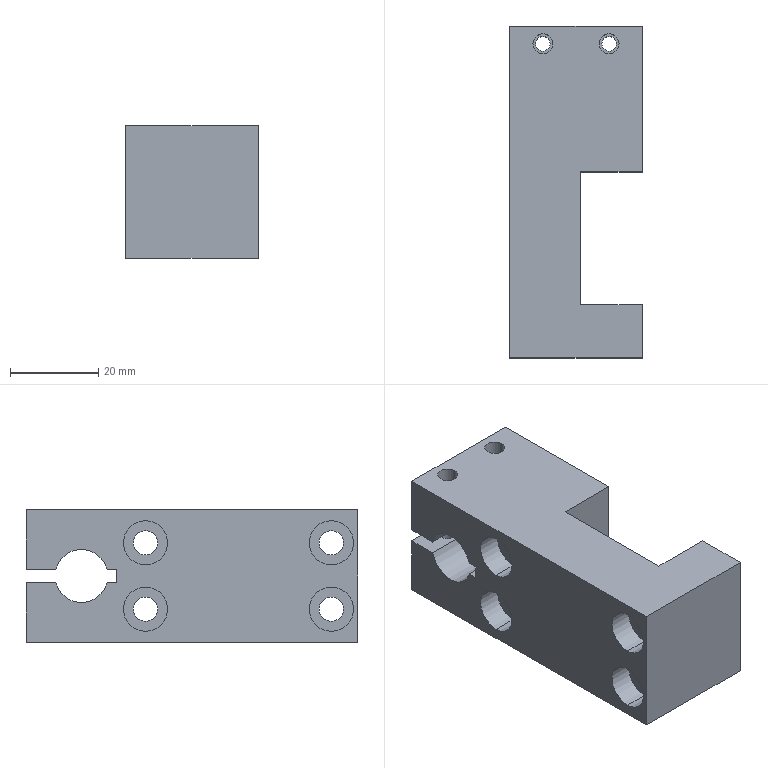Component | SolidWorks | XM-WST05-2005-1 | 1 solid | 46 faces | box 30 x 75 x 30 mm | volume 46036 mm3 | cylinder 26 | plane 20 | commonest cylinder face diameters 10 x8 5.5 x8 3.3 x4 4.5 x4 12 x2
build123d program:
from build123d import *

# Parameters (mm, degrees)
SKETCH1_W                                       = 30
SKETCH1_H                                       = 75
BOSS_EXTRUDE1_DEPTH                             = 15
SKETCH2_R                                       = 6
CUT_EXTRUDE1_DEPTH                              = 71.931
SKETCH4_W                                       = 3
SKETCH4_H                                       = 41
CUT_EXTRUDE3_DEPTH                              = 71.931
SKETCH11_W                                      = 30
SKETCH11_H                                      = 30
CUT_EXTRUDE6_DEPTH                              = 14
M5_HEX_SOCKET_HEAD_CAP_SCREW_CBORE2_D           = 5.5
M5_HEX_SOCKET_HEAD_CAP_SCREW_CBORE2_CBORE_D     = 10
M5_HEX_SOCKET_HEAD_CAP_SCREW_CBORE2_CBORE_DEPTH = 5.4
SKETCH17_R                                      = 2.25
CUT_EXTRUDE7_DEPTH                              = 13.5
M4_TAPPED_HOLE1_D                               = 3.3


with BuildPart() as part:
    # Sketch1 → Boss-Extrude1 (new, symmetric)
    with BuildSketch(Plane.XY):
        with Locations((0, 25)):
            Rectangle(SKETCH1_W, SKETCH1_H)
    extrude(amount=BOSS_EXTRUDE1_DEPTH, both=True)

    # Sketch2 → Cut-Extrude1 (cut, through all)
    with BuildSketch(Plane(origin=(15, 0, 0), x_dir=(0, 0, -1), z_dir=(1, 0, 0))):
        with Locations(Location((0, 50, 0), (0, 0, 90))):
            Circle(SKETCH2_R)
    extrude(amount=-CUT_EXTRUDE1_DEPTH, mode=Mode.SUBTRACT)

    # Sketch4 → Cut-Extrude3 (cut, through all)
    with BuildSketch(Plane(origin=(15, 0, 0), x_dir=(0, 0, -1), z_dir=(1, 0, 0))):
        with Locations((0, 62.5)):
            Rectangle(SKETCH4_W, SKETCH4_H)
    extrude(amount=-CUT_EXTRUDE3_DEPTH, mode=Mode.SUBTRACT)

    # Sketch11 → Cut-Extrude6 (cut)
    with BuildSketch(Plane(origin=(15, 0, 0), x_dir=(0, 0, -1), z_dir=(1, 0, 0))):
        with Locations((0, 14.5)):
            Rectangle(SKETCH11_W, SKETCH11_H)
    extrude(amount=-CUT_EXTRUDE6_DEPTH, mode=Mode.SUBTRACT)

    # M5 Hex Socket Head Cap Screw CBORE2 (through all)
    with Locations(Plane.ZY.offset(15)):
        with Locations((7.5, -6.5), (-7.5, -6.5), (7.5, 35.5), (-7.5, 35.5)):
            CounterBoreHole(M5_HEX_SOCKET_HEAD_CAP_SCREW_CBORE2_D / 2, M5_HEX_SOCKET_HEAD_CAP_SCREW_CBORE2_CBORE_D / 2, M5_HEX_SOCKET_HEAD_CAP_SCREW_CBORE2_CBORE_DEPTH)

    # Sketch17 → Cut-Extrude7 (cut)
    with BuildSketch(Plane.XY.offset(15)):
        with Locations((-7.5, 58.5)):
            Circle(SKETCH17_R)
        with Locations((7.5, 58.5)):
            Circle(SKETCH17_R)
    extrude(amount=-CUT_EXTRUDE7_DEPTH, mode=Mode.SUBTRACT)

    # M4 Tapped Hole1 (through all)
    with Locations(Plane.XY.offset(-1.5)):
        with Locations((-7.5, 58.5), (7.5, 58.5)):
            Hole(M4_TAPPED_HOLE1_D / 2)


solid = part.part

# Placed as in the assembly
solid = solid.moved(Location((-170.071, 34.169, 359.808), (0, 0, 0)))